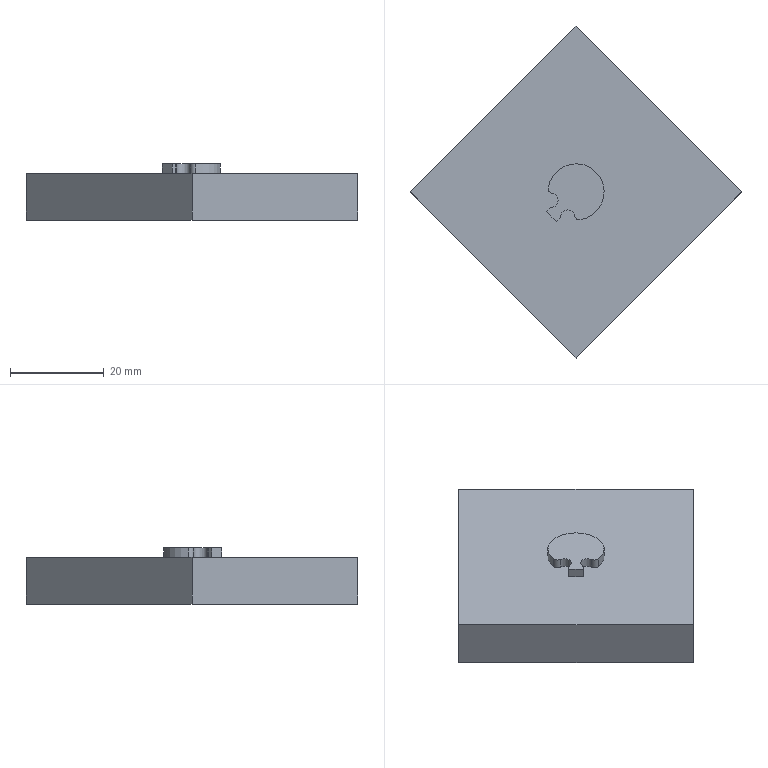CAM job | Mastercam | mm | 9 operations | part box 70.71 x 70.71 x 12
1. Facing | 24 - 100 平铣刀
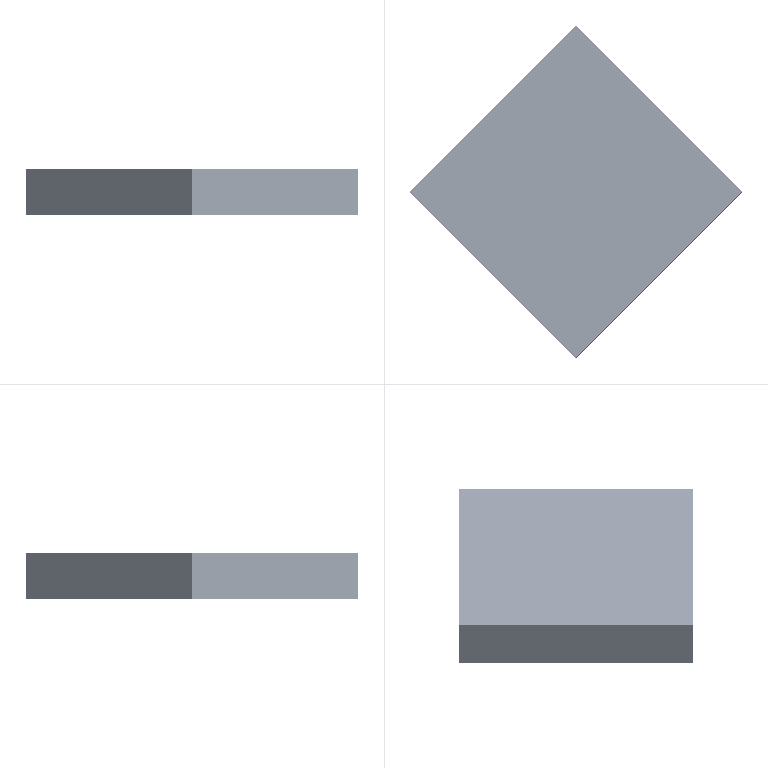2. Contour (Ramp) | 9 - 10 平铣刀
3. 2D High Speed (2D Area Mill) | 9 - 10 平铣刀
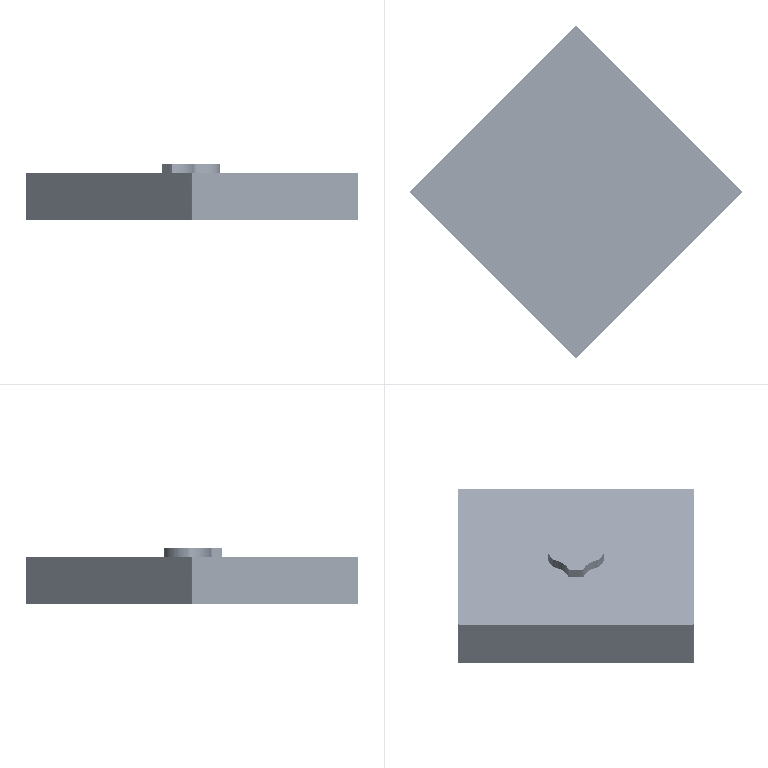4. Contour (2D) | 10 - 10 平铣刀
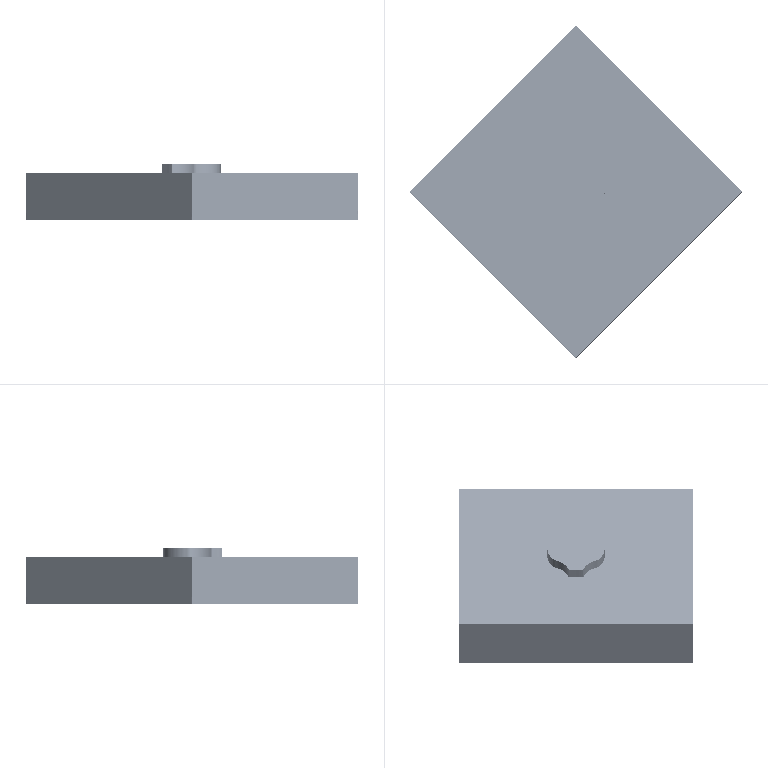5. 2D High Speed (2D Area Mill) | 10 - 10 平铣刀
6. Contour (Ramp) | 2 - 2 平铣刀
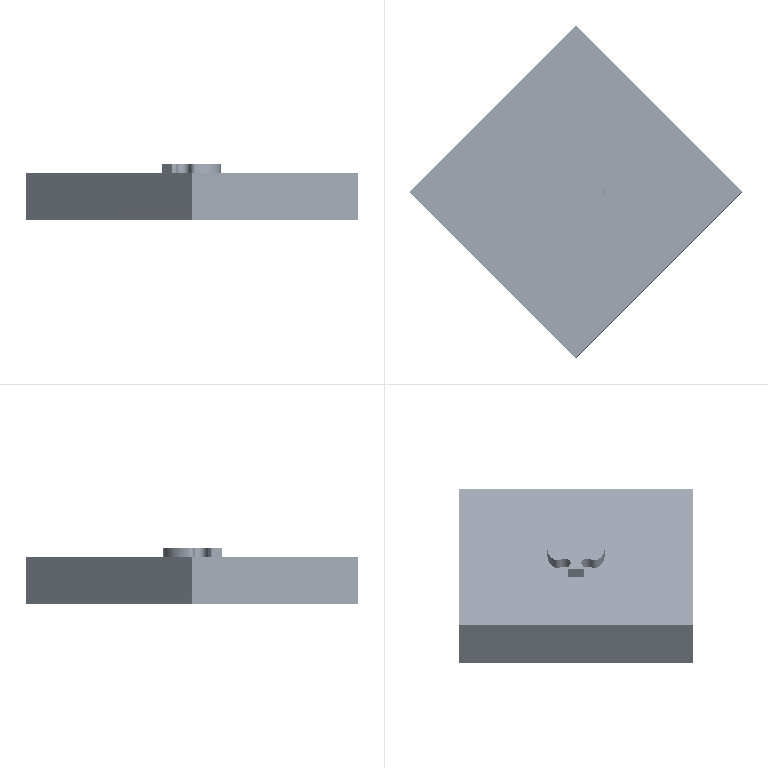7. Contour (2D) | 2 - 2 平铣刀
8. Contour (2D chamfer) | 5 - 4 倒角刀
9. Drill/Counterbore | 5 - 4 倒角刀